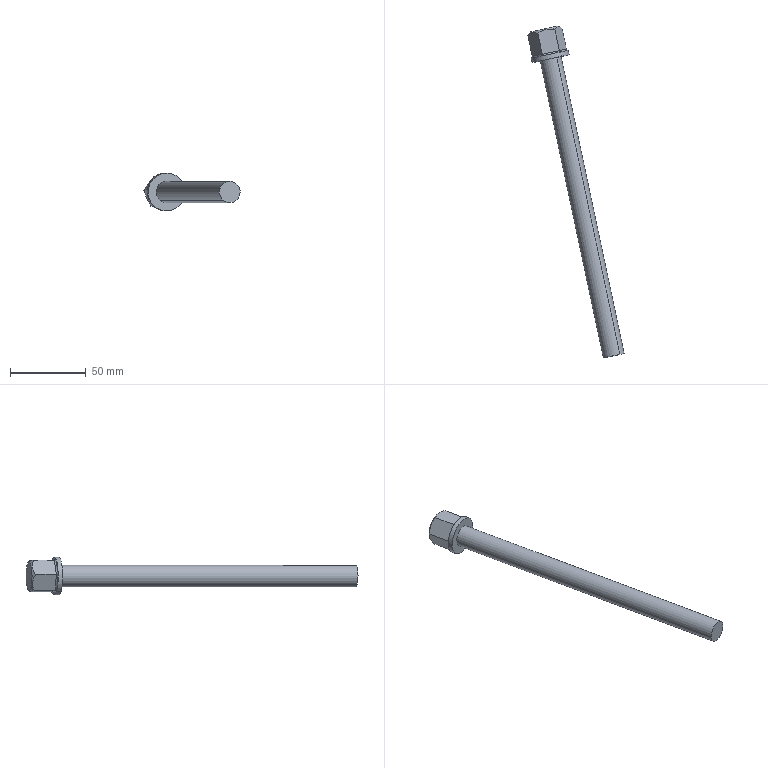Component | SolidWorks | 1Product25x2009.26-2 | 1 solid | 27 faces | volume 38128 mm3 | plane 15 | cylinder 10 | cone 2 | commonest cylinder face diameters 2 x6 14 x2 25 x2 | material AISI 1045 Steel, Cold Drawn